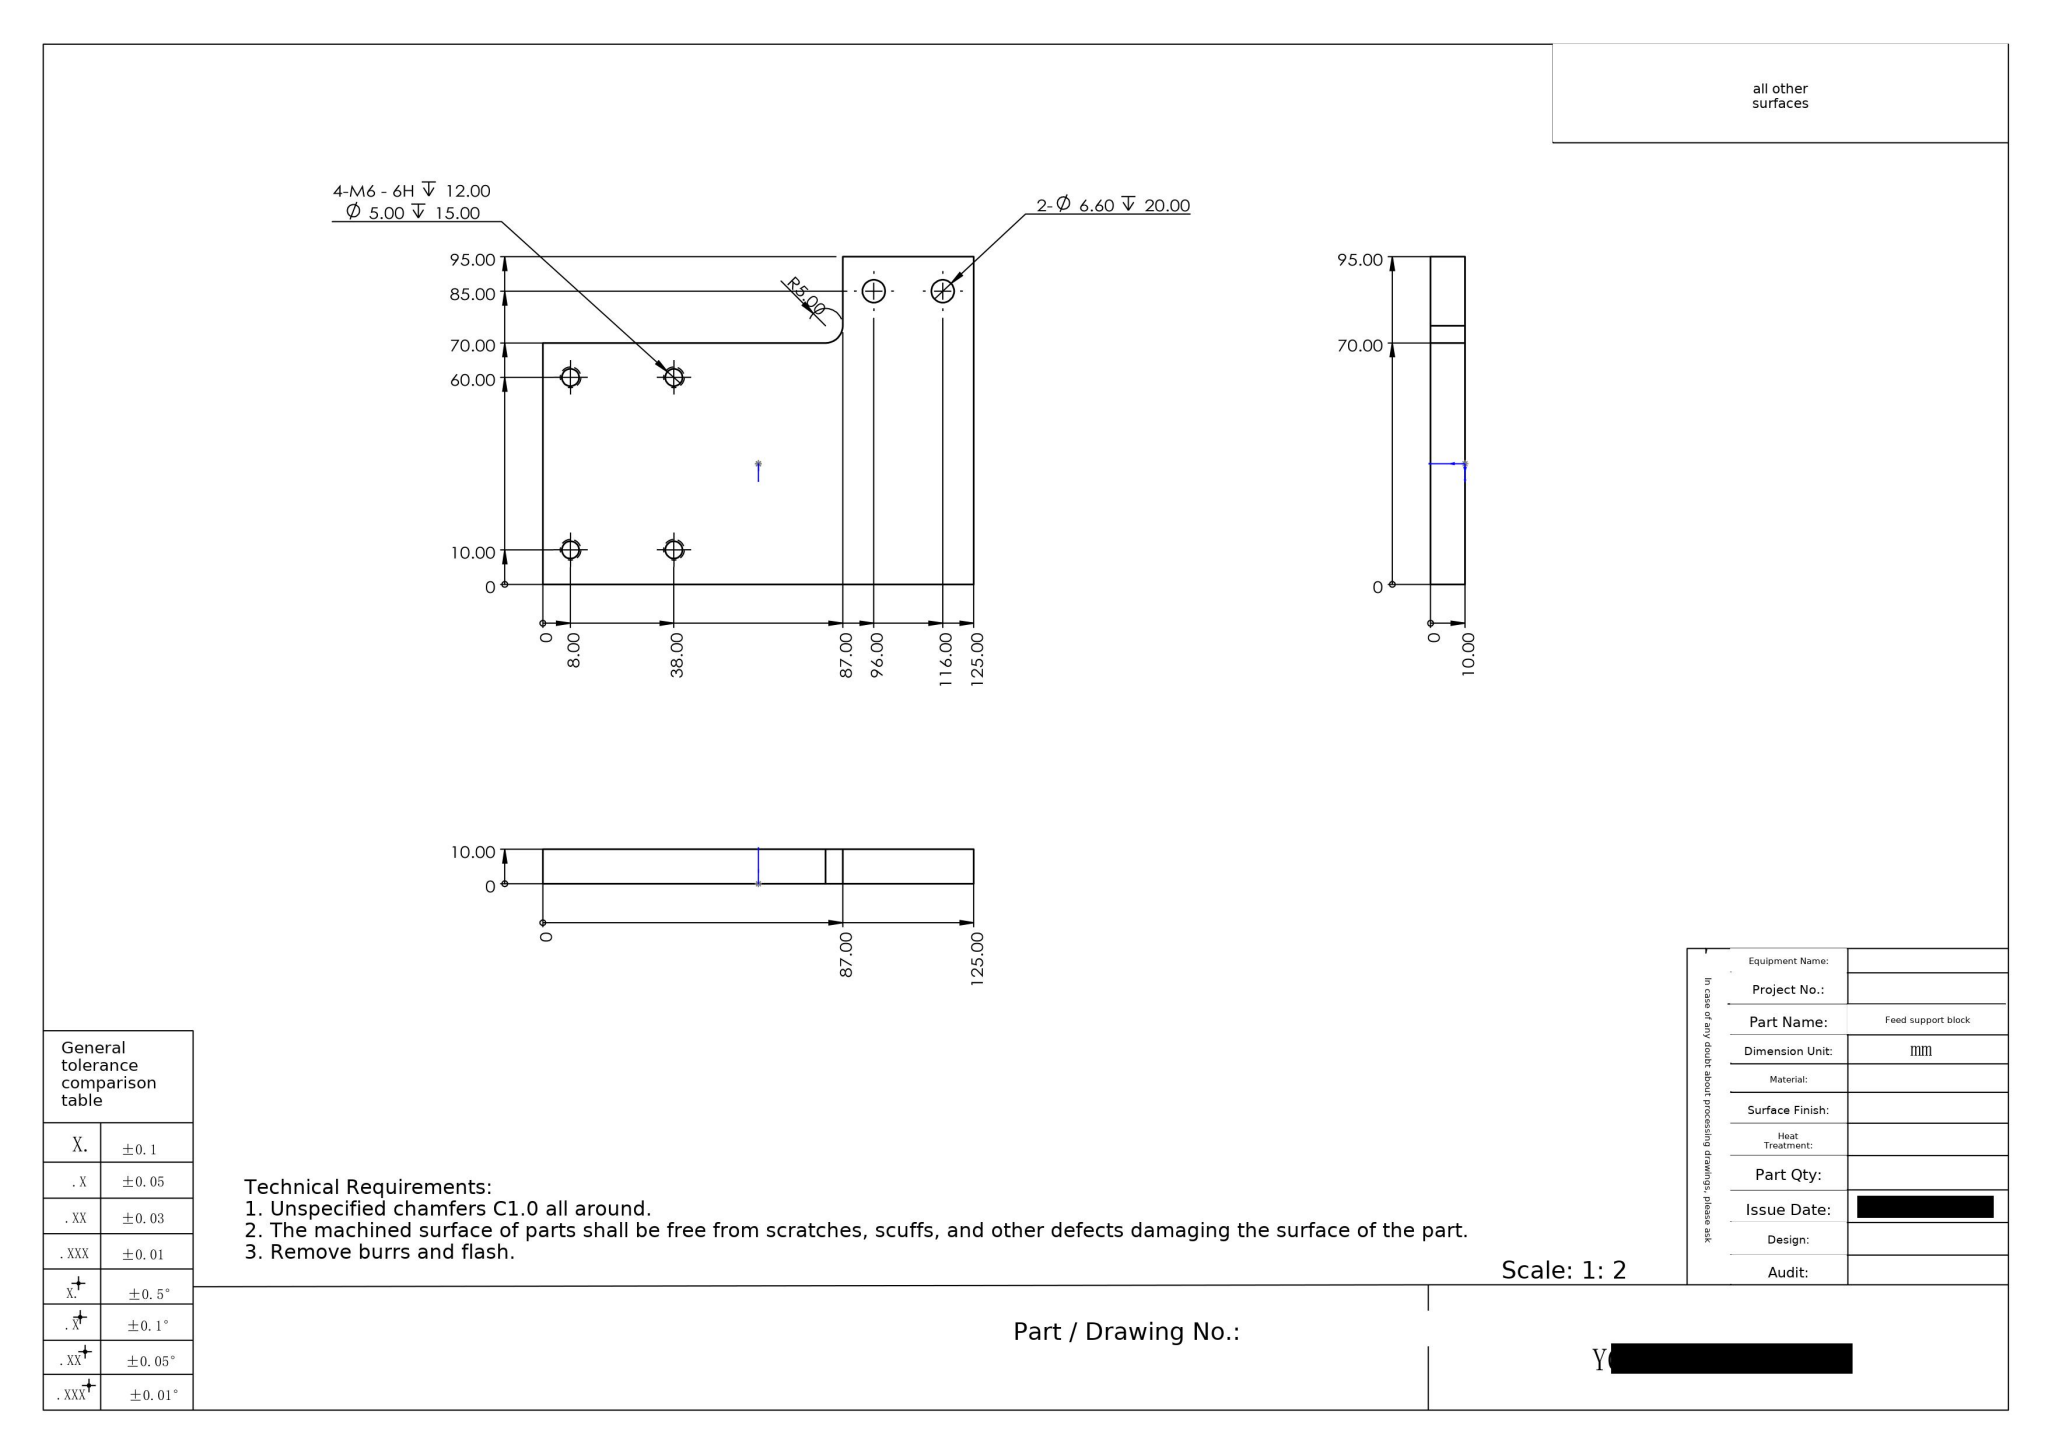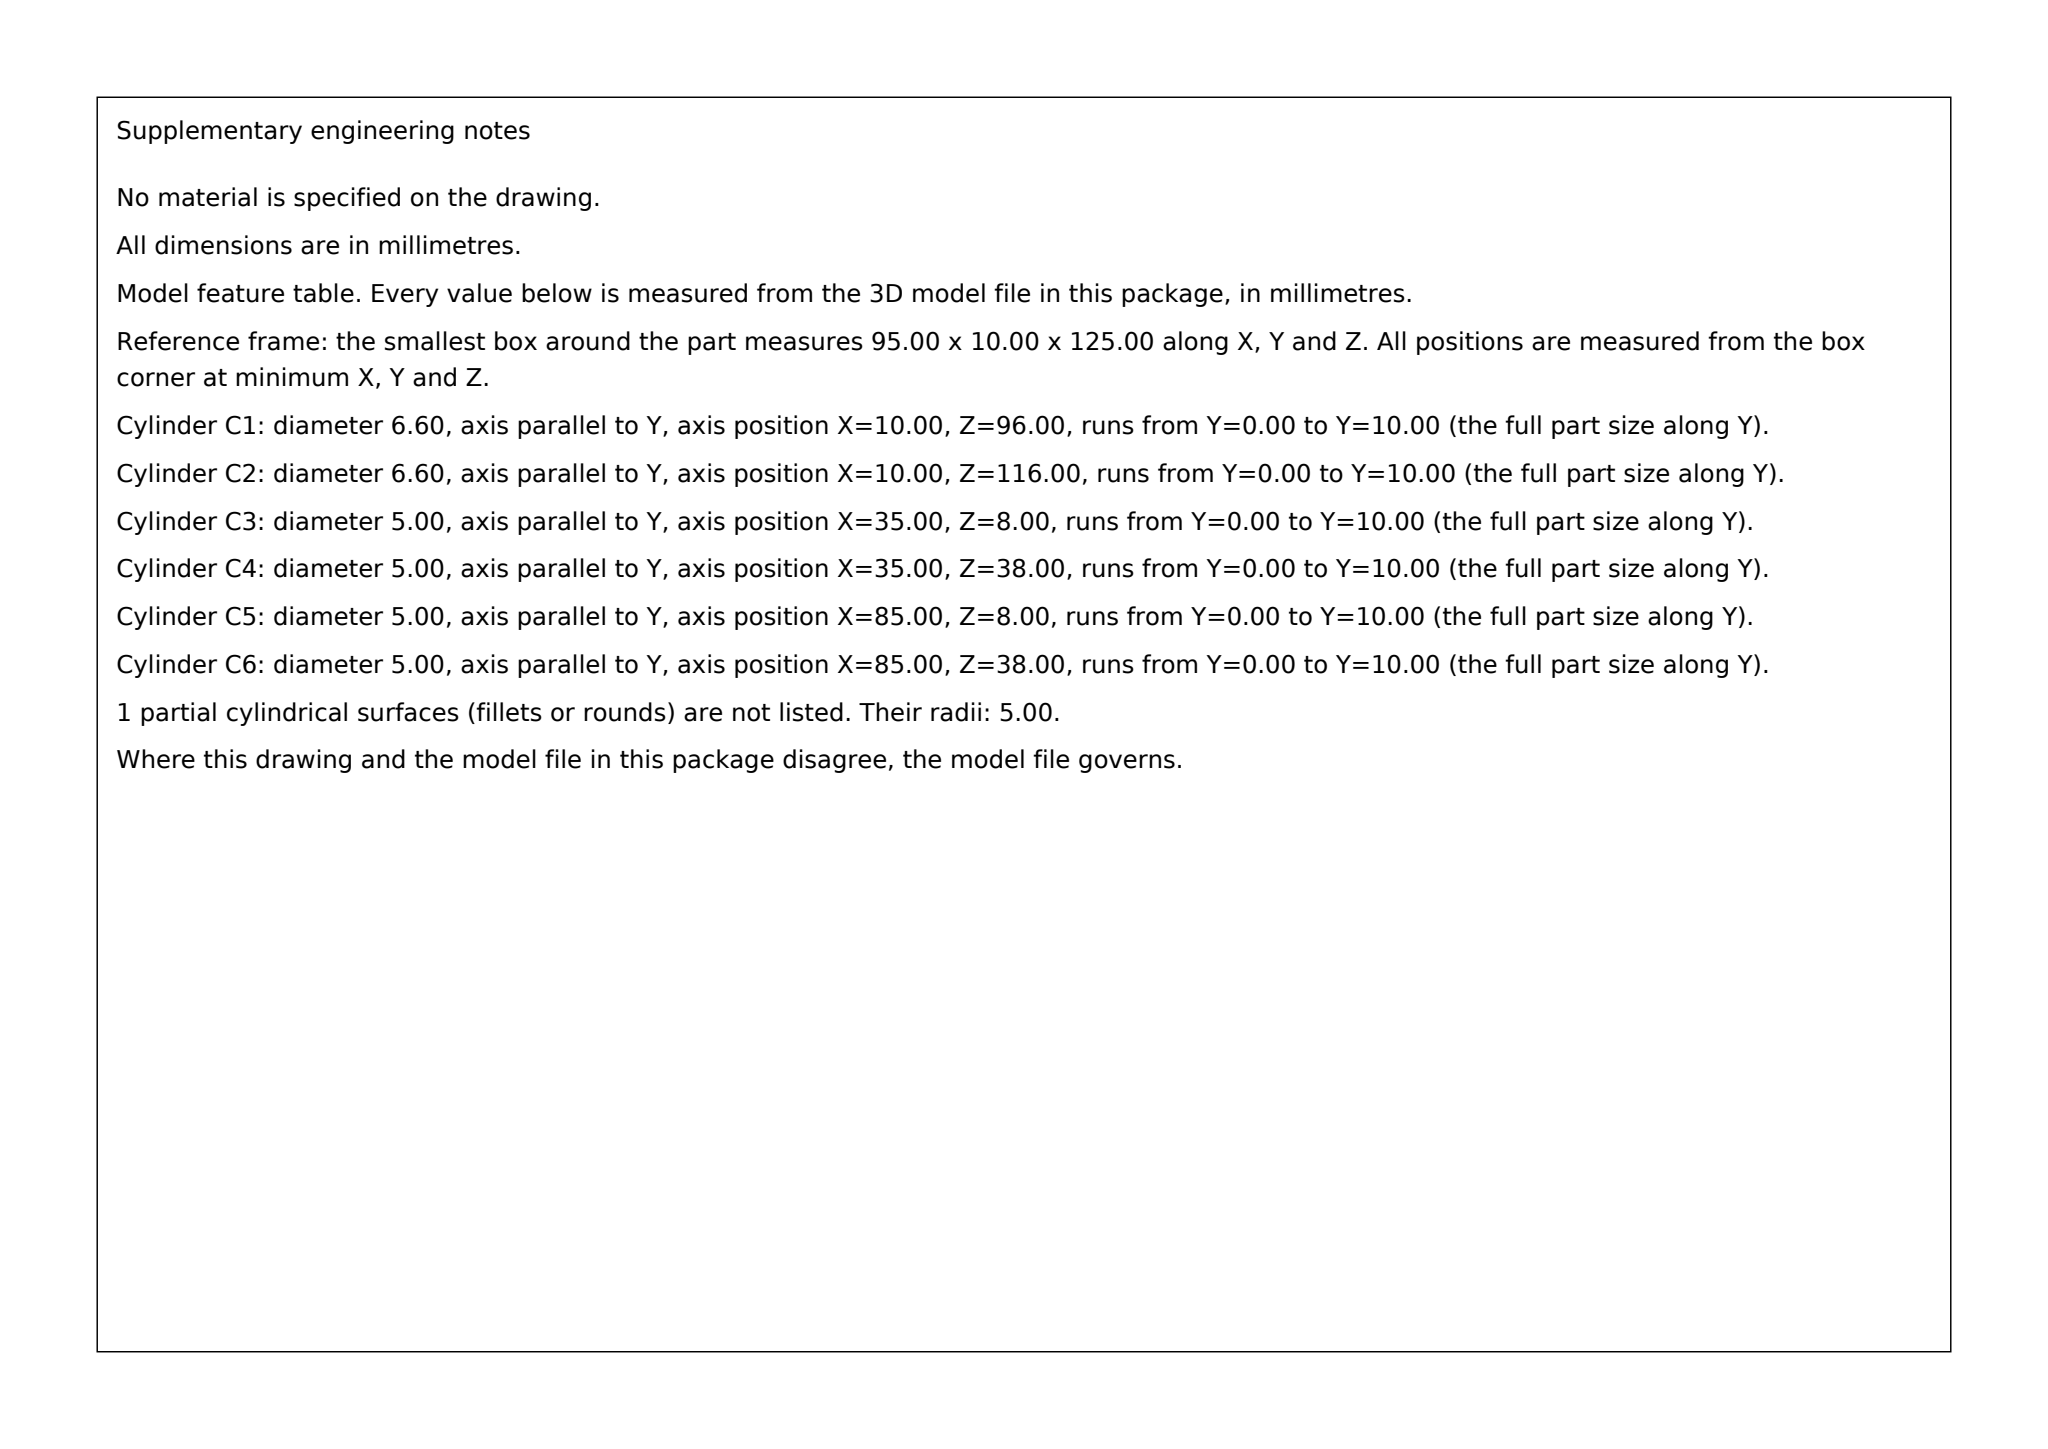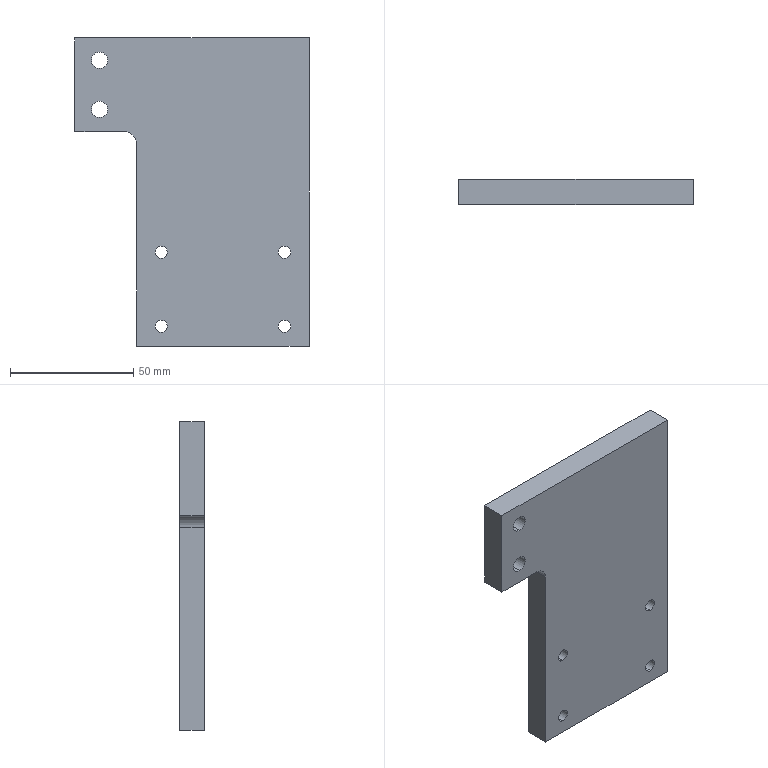Part | SolidWorks | mm | 1 solid | 21 faces | box 95 x 10 x 125 mm | volume 95584 mm3 | cylinder 13 | plane 8 | commonest cylinder face diameters 5 x8 6.6 x4 10 x1
build123d program:
from build123d import *

# Parameters (mm, degrees)
SKETCH1_W                = 70
SKETCH1_H                = 125
BOSS_EXTRUDE1_DEPTH      = 10
M6_TAPPED_HOLE1_D        = 5
M6_TAPPED_HOLE1_DEPTH    = 15
M6_TAPPED_HOLE1_TIP      = 1.502
SKETCH6_W                = 25
SKETCH6_H                = 38
BOSS_EXTRUDE2_DEPTH      = 10
M6_CLEARANCE_HOLE1_D     = 6.6
M6_CLEARANCE_HOLE1_DEPTH = 20
M6_CLEARANCE_HOLE1_TIP   = 1.983
FILLET1_R                = 5


with BuildPart() as part:
    # Sketch1 → Boss-Extrude1 (new body)
    with BuildSketch(Plane(origin=(0, 0, 0), x_dir=(1, 0, 0), z_dir=(0, 1, 0))):
        Rectangle(SKETCH1_W, SKETCH1_H)
    extrude(amount=BOSS_EXTRUDE1_DEPTH)

    # M6 Tapped Hole1
    with Locations(Plane(origin=(0, 10, 0), x_dir=(1, 0, 0), z_dir=(0, 1, 0))):
        with Locations((-25, 54.5), (25, 54.5), (-25, 24.5), (25, 24.5)):
            Hole(M6_TAPPED_HOLE1_D / 2, depth=M6_TAPPED_HOLE1_DEPTH)
            with Locations((0, 0, -(M6_TAPPED_HOLE1_DEPTH + M6_TAPPED_HOLE1_TIP / 2))):  # 118° drill point
                Cone(0, M6_TAPPED_HOLE1_D / 2, M6_TAPPED_HOLE1_TIP, mode=Mode.SUBTRACT)

    # Sketch6 → Boss-Extrude2 (add)
    with BuildSketch(Plane(origin=(0, 10, 0), x_dir=(1, 0, 0), z_dir=(0, 1, 0))):
        with Locations((-47.5, -43.5)):
            Rectangle(SKETCH6_W, SKETCH6_H)
    extrude(amount=-BOSS_EXTRUDE2_DEPTH)

    # M6 Clearance Hole1
    with Locations(Plane(origin=(0, 10, 0), x_dir=(1, 0, 0), z_dir=(0, 1, 0))):
        with Locations((-50, -33.5), (-50, -53.5)):
            Hole(M6_CLEARANCE_HOLE1_D / 2, depth=M6_CLEARANCE_HOLE1_DEPTH)
            with Locations((0, 0, -(M6_CLEARANCE_HOLE1_DEPTH + M6_CLEARANCE_HOLE1_TIP / 2))):  # 118° drill point
                Cone(0, M6_CLEARANCE_HOLE1_D / 2, M6_CLEARANCE_HOLE1_TIP, mode=Mode.SUBTRACT)

    # Fillet1
    fillet1_edges = [part.edges().sort_by_distance(p)[0] for p in [
        (-35, 5, 24.5),
    ]]
    fillet(fillet1_edges, radius=FILLET1_R)


solid = part.part
STEP:
#1=CARTESIAN_POINT('',(-50.,0.,30.2));
#2=VERTEX_POINT('',#1);
#3=CARTESIAN_POINT('',(-50.,0.,36.8));
#4=VERTEX_POINT('',#3);
#5=CARTESIAN_POINT('',(-50.,0.,33.5));
#6=DIRECTION('',(0.,1.,0.));
#7=DIRECTION('',(0.,0.,1.));
#8=AXIS2_PLACEMENT_3D('',#5,#6,#7);
#9=CIRCLE('',#8,3.3);
#10=EDGE_CURVE('',#2,#4,#9,.T.);
#11=ORIENTED_EDGE('',*,*,#10,.F.);
#12=CARTESIAN_POINT('',(-50.,10.,30.2));
#13=VERTEX_POINT('',#12);
#14=CARTESIAN_POINT('',(-50.,10.,30.2));
#15=DIRECTION('',(0.,1.,0.));
#16=VECTOR('',#15,1000.);
#17=LINE('',#14,#16);
#18=EDGE_CURVE('',#2,#13,#17,.T.);
#19=ORIENTED_EDGE('',*,*,#18,.T.);
#20=CARTESIAN_POINT('',(-50.,10.,36.8));
#21=VERTEX_POINT('',#20);
#22=CARTESIAN_POINT('',(-50.,10.,33.5));
#23=DIRECTION('',(0.,1.,0.));
#24=DIRECTION('',(0.,0.,1.));
#25=AXIS2_PLACEMENT_3D('',#22,#23,#24);
#26=CIRCLE('',#25,3.3);
#27=EDGE_CURVE('',#13,#21,#26,.T.);
#28=ORIENTED_EDGE('',*,*,#27,.T.);
#29=CARTESIAN_POINT('',(-50.,10.,36.8));
#30=DIRECTION('',(0.,1.,0.));
#31=VECTOR('',#30,1000.);
#32=LINE('',#29,#31);
#33=EDGE_CURVE('',#4,#21,#32,.T.);
#34=ORIENTED_EDGE('',*,*,#33,.F.);
#35=EDGE_LOOP('',(#11,#19,#28,#34));
#36=FACE_OUTER_BOUND('',#35,.T.);
#37=CARTESIAN_POINT('',(-50.,10.,33.5));
#38=DIRECTION('',(0.,1.,0.));
#39=DIRECTION('',(0.,0.,1.));
#40=AXIS2_PLACEMENT_3D('',#37,#38,#39);
#41=CYLINDRICAL_SURFACE('',#40,3.3);
#42=ADVANCED_FACE('',(#36),#41,.F.);
#43=CARTESIAN_POINT('',(-50.,0.,50.2));
#44=VERTEX_POINT('',#43);
#45=CARTESIAN_POINT('',(-50.,0.,56.8));
#46=VERTEX_POINT('',#45);
#47=CARTESIAN_POINT('',(-50.,0.,53.5));
#48=DIRECTION('',(0.,1.,0.));
#49=DIRECTION('',(0.,0.,1.));
#50=AXIS2_PLACEMENT_3D('',#47,#48,#49);
#51=CIRCLE('',#50,3.3);
#52=EDGE_CURVE('',#44,#46,#51,.T.);
#53=ORIENTED_EDGE('',*,*,#52,.F.);
#54=CARTESIAN_POINT('',(-50.,10.,50.2));
#55=VERTEX_POINT('',#54);
#56=CARTESIAN_POINT('',(-50.,10.,50.2));
#57=DIRECTION('',(0.,1.,0.));
#58=VECTOR('',#57,1000.);
#59=LINE('',#56,#58);
#60=EDGE_CURVE('',#44,#55,#59,.T.);
#61=ORIENTED_EDGE('',*,*,#60,.T.);
#62=CARTESIAN_POINT('',(-50.,10.,56.8));
#63=VERTEX_POINT('',#62);
#64=CARTESIAN_POINT('',(-50.,10.,53.5));
#65=DIRECTION('',(0.,1.,0.));
#66=DIRECTION('',(0.,0.,1.));
#67=AXIS2_PLACEMENT_3D('',#64,#65,#66);
#68=CIRCLE('',#67,3.3);
#69=EDGE_CURVE('',#55,#63,#68,.T.);
#70=ORIENTED_EDGE('',*,*,#69,.T.);
#71=CARTESIAN_POINT('',(-50.,10.,56.8));
#72=DIRECTION('',(0.,1.,0.));
#73=VECTOR('',#72,1000.);
#74=LINE('',#71,#73);
#75=EDGE_CURVE('',#46,#63,#74,.T.);
#76=ORIENTED_EDGE('',*,*,#75,.F.);
#77=EDGE_LOOP('',(#53,#61,#70,#76));
#78=FACE_OUTER_BOUND('',#77,.T.);
#79=CARTESIAN_POINT('',(-50.,10.,53.5));
#80=DIRECTION('',(0.,1.,0.));
#81=DIRECTION('',(0.,0.,1.));
#82=AXIS2_PLACEMENT_3D('',#79,#80,#81);
#83=CYLINDRICAL_SURFACE('',#82,3.3);
#84=ADVANCED_FACE('',(#78),#83,.F.);
#85=CARTESIAN_POINT('',(-25.,0.,-57.));
#86=VERTEX_POINT('',#85);
#87=CARTESIAN_POINT('',(-25.,0.,-52.));
#88=VERTEX_POINT('',#87);
#89=CARTESIAN_POINT('',(-25.,0.,-54.5));
#90=DIRECTION('',(0.,1.,0.));
#91=DIRECTION('',(0.,0.,1.));
#92=AXIS2_PLACEMENT_3D('',#89,#90,#91);
#93=CIRCLE('',#92,2.5);
#94=EDGE_CURVE('',#86,#88,#93,.T.);
#95=ORIENTED_EDGE('',*,*,#94,.F.);
#96=CARTESIAN_POINT('',(-25.,10.,-57.));
#97=VERTEX_POINT('',#96);
#98=CARTESIAN_POINT('',(-25.,10.,-57.));
#99=DIRECTION('',(0.,1.,0.));
#100=VECTOR('',#99,1000.);
#101=LINE('',#98,#100);
#102=EDGE_CURVE('',#86,#97,#101,.T.);
#103=ORIENTED_EDGE('',*,*,#102,.T.);
#104=CARTESIAN_POINT('',(-25.,10.,-52.));
#105=VERTEX_POINT('',#104);
#106=CARTESIAN_POINT('',(-25.,10.,-54.5));
#107=DIRECTION('',(0.,1.,0.));
#108=DIRECTION('',(0.,0.,1.));
#109=AXIS2_PLACEMENT_3D('',#106,#107,#108);
#110=CIRCLE('',#109,2.5);
#111=EDGE_CURVE('',#97,#105,#110,.T.);
#112=ORIENTED_EDGE('',*,*,#111,.T.);
#113=CARTESIAN_POINT('',(-25.,10.,-52.));
#114=DIRECTION('',(0.,1.,0.));
#115=VECTOR('',#114,1000.);
#116=LINE('',#113,#115);
#117=EDGE_CURVE('',#88,#105,#116,.T.);
#118=ORIENTED_EDGE('',*,*,#117,.F.);
#119=EDGE_LOOP('',(#95,#103,#112,#118));
#120=FACE_OUTER_BOUND('',#119,.T.);
#121=CARTESIAN_POINT('',(-25.,10.,-54.5));
#122=DIRECTION('',(0.,1.,0.));
#123=DIRECTION('',(0.,0.,1.));
#124=AXIS2_PLACEMENT_3D('',#121,#122,#123);
#125=CYLINDRICAL_SURFACE('',#124,2.5);
#126=ADVANCED_FACE('',(#120),#125,.F.);
#127=CARTESIAN_POINT('',(25.,0.,-57.));
#128=VERTEX_POINT('',#127);
#129=CARTESIAN_POINT('',(25.,0.,-52.));
#130=VERTEX_POINT('',#129);
#131=CARTESIAN_POINT('',(25.,0.,-54.5));
#132=DIRECTION('',(0.,1.,0.));
#133=DIRECTION('',(0.,0.,1.));
#134=AXIS2_PLACEMENT_3D('',#131,#132,#133);
#135=CIRCLE('',#134,2.5);
#136=EDGE_CURVE('',#128,#130,#135,.T.);
#137=ORIENTED_EDGE('',*,*,#136,.F.);
#138=CARTESIAN_POINT('',(25.,10.,-57.));
#139=VERTEX_POINT('',#138);
#140=CARTESIAN_POINT('',(25.,10.,-57.));
#141=DIRECTION('',(0.,1.,0.));
#142=VECTOR('',#141,1000.);
#143=LINE('',#140,#142);
#144=EDGE_CURVE('',#128,#139,#143,.T.);
#145=ORIENTED_EDGE('',*,*,#144,.T.);
#146=CARTESIAN_POINT('',(25.,10.,-52.));
#147=VERTEX_POINT('',#146);
#148=CARTESIAN_POINT('',(25.,10.,-54.5));
#149=DIRECTION('',(0.,1.,0.));
#150=DIRECTION('',(0.,0.,1.));
#151=AXIS2_PLACEMENT_3D('',#148,#149,#150);
#152=CIRCLE('',#151,2.5);
#153=EDGE_CURVE('',#139,#147,#152,.T.);
#154=ORIENTED_EDGE('',*,*,#153,.T.);
#155=CARTESIAN_POINT('',(25.,10.,-52.));
#156=DIRECTION('',(0.,1.,0.));
#157=VECTOR('',#156,1000.);
#158=LINE('',#155,#157);
#159=EDGE_CURVE('',#130,#147,#158,.T.);
#160=ORIENTED_EDGE('',*,*,#159,.F.);
#161=EDGE_LOOP('',(#137,#145,#154,#160));
#162=FACE_OUTER_BOUND('',#161,.T.);
#163=CARTESIAN_POINT('',(25.,10.,-54.5));
#164=DIRECTION('',(0.,1.,0.));
#165=DIRECTION('',(0.,0.,1.));
#166=AXIS2_PLACEMENT_3D('',#163,#164,#165);
#167=CYLINDRICAL_SURFACE('',#166,2.5);
#168=ADVANCED_FACE('',(#162),#167,.F.);
#169=CARTESIAN_POINT('',(-25.,0.,-27.));
#170=VERTEX_POINT('',#169);
#171=CARTESIAN_POINT('',(-25.,0.,-22.));
#172=VERTEX_POINT('',#171);
#173=CARTESIAN_POINT('',(-25.,0.,-24.5));
#174=DIRECTION('',(0.,1.,0.));
#175=DIRECTION('',(0.,0.,1.));
#176=AXIS2_PLACEMENT_3D('',#173,#174,#175);
#177=CIRCLE('',#176,2.5);
#178=EDGE_CURVE('',#170,#172,#177,.T.);
#179=ORIENTED_EDGE('',*,*,#178,.F.);
#180=CARTESIAN_POINT('',(-25.,10.,-27.));
#181=VERTEX_POINT('',#180);
#182=CARTESIAN_POINT('',(-25.,10.,-27.));
#183=DIRECTION('',(0.,1.,0.));
#184=VECTOR('',#183,1000.);
#185=LINE('',#182,#184);
#186=EDGE_CURVE('',#170,#181,#185,.T.);
#187=ORIENTED_EDGE('',*,*,#186,.T.);
#188=CARTESIAN_POINT('',(-25.,10.,-22.));
#189=VERTEX_POINT('',#188);
#190=CARTESIAN_POINT('',(-25.,10.,-24.5));
#191=DIRECTION('',(0.,1.,0.));
#192=DIRECTION('',(0.,0.,1.));
#193=AXIS2_PLACEMENT_3D('',#190,#191,#192);
#194=CIRCLE('',#193,2.5);
#195=EDGE_CURVE('',#181,#189,#194,.T.);
#196=ORIENTED_EDGE('',*,*,#195,.T.);
#197=CARTESIAN_POINT('',(-25.,10.,-22.));
#198=DIRECTION('',(0.,1.,0.));
#199=VECTOR('',#198,1000.);
#200=LINE('',#197,#199);
#201=EDGE_CURVE('',#172,#189,#200,.T.);
#202=ORIENTED_EDGE('',*,*,#201,.F.);
#203=EDGE_LOOP('',(#179,#187,#196,#202));
#204=FACE_OUTER_BOUND('',#203,.T.);
#205=CARTESIAN_POINT('',(-25.,10.,-24.5));
#206=DIRECTION('',(0.,1.,0.));
#207=DIRECTION('',(0.,0.,1.));
#208=AXIS2_PLACEMENT_3D('',#205,#206,#207);
#209=CYLINDRICAL_SURFACE('',#208,2.5);
#210=ADVANCED_FACE('',(#204),#209,.F.);
#211=CARTESIAN_POINT('',(25.,0.,-27.));
#212=VERTEX_POINT('',#211);
#213=CARTESIAN_POINT('',(25.,0.,-22.));
#214=VERTEX_POINT('',#213);
#215=CARTESIAN_POINT('',(25.,0.,-24.5));
#216=DIRECTION('',(0.,1.,0.));
#217=DIRECTION('',(0.,0.,1.));
#218=AXIS2_PLACEMENT_3D('',#215,#216,#217);
#219=CIRCLE('',#218,2.5);
#220=EDGE_CURVE('',#212,#214,#219,.T.);
#221=ORIENTED_EDGE('',*,*,#220,.F.);
#222=CARTESIAN_POINT('',(25.,10.,-27.));
#223=VERTEX_POINT('',#222);
#224=CARTESIAN_POINT('',(25.,10.,-27.));
#225=DIRECTION('',(0.,1.,0.));
#226=VECTOR('',#225,1000.);
#227=LINE('',#224,#226);
#228=EDGE_CURVE('',#212,#223,#227,.T.);
#229=ORIENTED_EDGE('',*,*,#228,.T.);
#230=CARTESIAN_POINT('',(25.,10.,-22.));
#231=VERTEX_POINT('',#230);
#232=CARTESIAN_POINT('',(25.,10.,-24.5));
#233=DIRECTION('',(0.,1.,0.));
#234=DIRECTION('',(0.,0.,1.));
#235=AXIS2_PLACEMENT_3D('',#232,#233,#234);
#236=CIRCLE('',#235,2.5);
#237=EDGE_CURVE('',#223,#231,#236,.T.);
#238=ORIENTED_EDGE('',*,*,#237,.T.);
#239=CARTESIAN_POINT('',(25.,10.,-22.));
#240=DIRECTION('',(0.,1.,0.));
#241=VECTOR('',#240,1000.);
#242=LINE('',#239,#241);
#243=EDGE_CURVE('',#214,#231,#242,.T.);
#244=ORIENTED_EDGE('',*,*,#243,.F.);
#245=EDGE_LOOP('',(#221,#229,#238,#244));
#246=FACE_OUTER_BOUND('',#245,.T.);
#247=CARTESIAN_POINT('',(25.,10.,-24.5));
#248=DIRECTION('',(0.,1.,0.));
#249=DIRECTION('',(0.,0.,1.));
#250=AXIS2_PLACEMENT_3D('',#247,#248,#249);
#251=CYLINDRICAL_SURFACE('',#250,2.5);
#252=ADVANCED_FACE('',(#246),#251,.F.);
#253=CARTESIAN_POINT('',(-35.,0.,-62.5));
#254=VERTEX_POINT('',#253);
#255=CARTESIAN_POINT('',(-35.,0.,19.5));
#256=VERTEX_POINT('',#255);
#257=CARTESIAN_POINT('',(-35.,0.,-62.5));
#258=DIRECTION('',(0.,0.,1.));
#259=VECTOR('',#258,1000.);
#260=LINE('',#257,#259);
#261=EDGE_CURVE('',#254,#256,#260,.T.);
#262=ORIENTED_EDGE('',*,*,#261,.T.);
#263=CARTESIAN_POINT('',(-35.,10.,19.5));
#264=VERTEX_POINT('',#263);
#265=CARTESIAN_POINT('',(-35.,10.,19.5));
#266=DIRECTION('',(0.,1.,0.));
#267=VECTOR('',#266,1000.);
#268=LINE('',#265,#267);
#269=EDGE_CURVE('',#256,#264,#268,.T.);
#270=ORIENTED_EDGE('',*,*,#269,.T.);
#271=CARTESIAN_POINT('',(-35.,10.,-62.5));
#272=VERTEX_POINT('',#271);
#273=CARTESIAN_POINT('',(-35.,10.,-62.5));
#274=DIRECTION('',(0.,0.,1.));
#275=VECTOR('',#274,1000.);
#276=LINE('',#273,#275);
#277=EDGE_CURVE('',#272,#264,#276,.T.);
#278=ORIENTED_EDGE('',*,*,#277,.F.);
#279=CARTESIAN_POINT('',(-35.,10.,-62.5));
#280=DIRECTION('',(0.,-1.,0.));
#281=VECTOR('',#280,1000.);
#282=LINE('',#279,#281);
#283=EDGE_CURVE('',#272,#254,#282,.T.);
#284=ORIENTED_EDGE('',*,*,#283,.T.);
#285=EDGE_LOOP('',(#262,#270,#278,#284));
#286=FACE_OUTER_BOUND('',#285,.T.);
#287=CARTESIAN_POINT('',(-35.,10.,-62.5));
#288=DIRECTION('',(1.,0.,-0.));
#289=DIRECTION('',(-0.,0.,-1.));
#290=AXIS2_PLACEMENT_3D('',#287,#288,#289);
#291=PLANE('',#290);
#292=ADVANCED_FACE('',(#286),#291,.F.);
#293=CARTESIAN_POINT('',(-60.,0.,62.5));
#294=VERTEX_POINT('',#293);
#295=CARTESIAN_POINT('',(35.,0.,62.5));
#296=VERTEX_POINT('',#295);
#297=CARTESIAN_POINT('',(-35.,0.,62.5));
#298=DIRECTION('',(1.,0.,0.));
#299=VECTOR('',#298,1000.);
#300=LINE('',#297,#299);
#301=EDGE_CURVE('',#294,#296,#300,.T.);
#302=ORIENTED_EDGE('',*,*,#301,.T.);
#303=CARTESIAN_POINT('',(35.,10.,62.5));
#304=VERTEX_POINT('',#303);
#305=CARTESIAN_POINT('',(35.,10.,62.5));
#306=DIRECTION('',(0.,-1.,0.));
#307=VECTOR('',#306,1000.);
#308=LINE('',#305,#307);
#309=EDGE_CURVE('',#304,#296,#308,.T.);
#310=ORIENTED_EDGE('',*,*,#309,.F.);
#311=CARTESIAN_POINT('',(-60.,10.,62.5));
#312=VERTEX_POINT('',#311);
#313=CARTESIAN_POINT('',(-35.,10.,62.5));
#314=DIRECTION('',(1.,0.,0.));
#315=VECTOR('',#314,1000.);
#316=LINE('',#313,#315);
#317=EDGE_CURVE('',#312,#304,#316,.T.);
#318=ORIENTED_EDGE('',*,*,#317,.F.);
#319=CARTESIAN_POINT('',(-60.,-45.486,62.5));
#320=DIRECTION('',(0.,1.,0.));
#321=VECTOR('',#320,1000.);
#322=LINE('',#319,#321);
#323=EDGE_CURVE('',#294,#312,#322,.T.);
#324=ORIENTED_EDGE('',*,*,#323,.F.);
#325=EDGE_LOOP('',(#302,#310,#318,#324));
#326=FACE_OUTER_BOUND('',#325,.T.);
#327=CARTESIAN_POINT('',(-35.,10.,62.5));
#328=DIRECTION('',(0.,0.,-1.));
#329=DIRECTION('',(-1.,0.,0.));
#330=AXIS2_PLACEMENT_3D('',#327,#328,#329);
#331=PLANE('',#330);
#332=ADVANCED_FACE('',(#326),#331,.F.);
#333=CARTESIAN_POINT('',(35.,0.,-62.5));
#334=VERTEX_POINT('',#333);
#335=CARTESIAN_POINT('',(35.,0.,-62.5));
#336=DIRECTION('',(0.,0.,1.));
#337=VECTOR('',#336,1000.);
#338=LINE('',#335,#337);
#339=EDGE_CURVE('',#334,#296,#338,.T.);
#340=ORIENTED_EDGE('',*,*,#339,.F.);
#341=CARTESIAN_POINT('',(35.,10.,-62.5));
#342=VERTEX_POINT('',#341);
#343=CARTESIAN_POINT('',(35.,10.,-62.5));
#344=DIRECTION('',(0.,-1.,0.));
#345=VECTOR('',#344,1000.);
#346=LINE('',#343,#345);
#347=EDGE_CURVE('',#342,#334,#346,.T.);
#348=ORIENTED_EDGE('',*,*,#347,.F.);
#349=CARTESIAN_POINT('',(35.,10.,-62.5));
#350=DIRECTION('',(0.,0.,1.));
#351=VECTOR('',#350,1000.);
#352=LINE('',#349,#351);
#353=EDGE_CURVE('',#342,#304,#352,.T.);
#354=ORIENTED_EDGE('',*,*,#353,.T.);
#355=ORIENTED_EDGE('',*,*,#309,.T.);
#356=EDGE_LOOP('',(#340,#348,#354,#355));
#357=FACE_OUTER_BOUND('',#356,.T.);
#358=CARTESIAN_POINT('',(35.,10.,-62.5));
#359=DIRECTION('',(1.,0.,-0.));
#360=DIRECTION('',(-0.,0.,-1.));
#361=AXIS2_PLACEMENT_3D('',#358,#359,#360);
#362=PLANE('',#361);
#363=ADVANCED_FACE('',(#357),#362,.T.);
#364=CARTESIAN_POINT('',(-35.,0.,-62.5));
#365=DIRECTION('',(1.,0.,0.));
#366=VECTOR('',#365,1000.);
#367=LINE('',#364,#366);
#368=EDGE_CURVE('',#254,#334,#367,.T.);
#369=ORIENTED_EDGE('',*,*,#368,.F.);
#370=ORIENTED_EDGE('',*,*,#283,.F.);
#371=CARTESIAN_POINT('',(-35.,10.,-62.5));
#372=DIRECTION('',(1.,0.,0.));
#373=VECTOR('',#372,1000.);
#374=LINE('',#371,#373);
#375=EDGE_CURVE('',#272,#342,#374,.T.);
#376=ORIENTED_EDGE('',*,*,#375,.T.);
#377=ORIENTED_EDGE('',*,*,#347,.T.);
#378=EDGE_LOOP('',(#369,#370,#376,#377));
#379=FACE_OUTER_BOUND('',#378,.T.);
#380=CARTESIAN_POINT('',(-35.,10.,-62.5));
#381=DIRECTION('',(0.,0.,-1.));
#382=DIRECTION('',(-1.,0.,0.));
#383=AXIS2_PLACEMENT_3D('',#380,#381,#382);
#384=PLANE('',#383);
#385=ADVANCED_FACE('',(#379),#384,.T.);
#386=CARTESIAN_POINT('',(-50.,10.,33.5));
#387=DIRECTION('',(0.,1.,0.));
#388=DIRECTION('',(0.,0.,1.));
#389=AXIS2_PLACEMENT_3D('',#386,#387,#388);
#390=CIRCLE('',#389,3.3);
#391=EDGE_CURVE('',#21,#13,#390,.T.);
#392=ORIENTED_EDGE('',*,*,#391,.F.);
#393=ORIENTED_EDGE('',*,*,#27,.F.);
#394=EDGE_LOOP('',(#392,#393));
#395=FACE_BOUND('',#394,.T.);
#396=CARTESIAN_POINT('',(-50.,10.,53.5));
#397=DIRECTION('',(0.,1.,0.));
#398=DIRECTION('',(0.,0.,1.));
#399=AXIS2_PLACEMENT_3D('',#396,#397,#398);
#400=CIRCLE('',#399,3.3);
#401=EDGE_CURVE('',#63,#55,#400,.T.);
#402=ORIENTED_EDGE('',*,*,#401,.F.);
#403=ORIENTED_EDGE('',*,*,#69,.F.);
#404=EDGE_LOOP('',(#402,#403));
#405=FACE_BOUND('',#404,.T.);
#406=CARTESIAN_POINT('',(-25.,10.,-54.5));
#407=DIRECTION('',(0.,1.,0.));
#408=DIRECTION('',(0.,0.,1.));
#409=AXIS2_PLACEMENT_3D('',#406,#407,#408);
#410=CIRCLE('',#409,2.5);
#411=EDGE_CURVE('',#105,#97,#410,.T.);
#412=ORIENTED_EDGE('',*,*,#411,.F.);
#413=ORIENTED_EDGE('',*,*,#111,.F.);
#414=EDGE_LOOP('',(#412,#413));
#415=FACE_BOUND('',#414,.T.);
#416=CARTESIAN_POINT('',(25.,10.,-54.5));
#417=DIRECTION('',(0.,1.,0.));
#418=DIRECTION('',(0.,0.,1.));
#419=AXIS2_PLACEMENT_3D('',#416,#417,#418);
#420=CIRCLE('',#419,2.5);
#421=EDGE_CURVE('',#147,#139,#420,.T.);
#422=ORIENTED_EDGE('',*,*,#421,.F.);
#423=ORIENTED_EDGE('',*,*,#153,.F.);
#424=EDGE_LOOP('',(#422,#423));
#425=FACE_BOUND('',#424,.T.);
#426=CARTESIAN_POINT('',(-25.,10.,-24.5));
#427=DIRECTION('',(0.,1.,0.));
#428=DIRECTION('',(0.,0.,1.));
#429=AXIS2_PLACEMENT_3D('',#426,#427,#428);
#430=CIRCLE('',#429,2.5);
#431=EDGE_CURVE('',#189,#181,#430,.T.);
#432=ORIENTED_EDGE('',*,*,#431,.F.);
#433=ORIENTED_EDGE('',*,*,#195,.F.);
#434=EDGE_LOOP('',(#432,#433));
#435=FACE_BOUND('',#434,.T.);
#436=CARTESIAN_POINT('',(25.,10.,-24.5));
#437=DIRECTION('',(0.,1.,0.));
#438=DIRECTION('',(0.,0.,1.));
#439=AXIS2_PLACEMENT_3D('',#436,#437,#438);
#440=CIRCLE('',#439,2.5);
#441=EDGE_CURVE('',#231,#223,#440,.T.);
#442=ORIENTED_EDGE('',*,*,#441,.F.);
#443=ORIENTED_EDGE('',*,*,#237,.F.);
#444=EDGE_LOOP('',(#442,#443));
#445=FACE_BOUND('',#444,.T.);
#446=ORIENTED_EDGE('',*,*,#277,.T.);
#447=CARTESIAN_POINT('',(-40.,10.,24.5));
#448=VERTEX_POINT('',#447);
#449=CARTESIAN_POINT('',(-40.,10.,19.5));
#450=DIRECTION('',(0.,-1.,0.));
#451=DIRECTION('',(0.,0.,1.));
#452=AXIS2_PLACEMENT_3D('',#449,#450,#451);
#453=CIRCLE('',#452,5.);
#454=EDGE_CURVE('',#264,#448,#453,.T.);
#455=ORIENTED_EDGE('',*,*,#454,.T.);
#456=CARTESIAN_POINT('',(-60.,10.,24.5));
#457=VERTEX_POINT('',#456);
#458=CARTESIAN_POINT('',(-35.,10.,24.5));
#459=DIRECTION('',(-1.,0.,0.));
#460=VECTOR('',#459,1000.);
#461=LINE('',#458,#460);
#462=EDGE_CURVE('',#448,#457,#461,.T.);
#463=ORIENTED_EDGE('',*,*,#462,.T.);
#464=CARTESIAN_POINT('',(-60.,10.,24.5));
#465=DIRECTION('',(0.,0.,1.));
#466=VECTOR('',#465,1000.);
#467=LINE('',#464,#466);
#468=EDGE_CURVE('',#457,#312,#467,.T.);
#469=ORIENTED_EDGE('',*,*,#468,.T.);
#470=ORIENTED_EDGE('',*,*,#317,.T.);
#471=ORIENTED_EDGE('',*,*,#353,.F.);
#472=ORIENTED_EDGE('',*,*,#375,.F.);
#473=EDGE_LOOP('',(#446,#455,#463,#469,#470,#471,#472));
#474=FACE_OUTER_BOUND('',#473,.T.);
#475=CARTESIAN_POINT('',(0.,10.,0.));
#476=DIRECTION('',(0.,1.,0.));
#477=DIRECTION('',(0.,0.,1.));
#478=AXIS2_PLACEMENT_3D('',#475,#476,#477);
#479=PLANE('',#478);
#480=ADVANCED_FACE('',(#395,#405,#415,#425,#435,#445,#474),#479,.T.);
#481=CARTESIAN_POINT('',(-50.,0.,33.5));
#482=DIRECTION('',(0.,1.,0.));
#483=DIRECTION('',(0.,0.,1.));
#484=AXIS2_PLACEMENT_3D('',#481,#482,#483);
#485=CIRCLE('',#484,3.3);
#486=EDGE_CURVE('',#4,#2,#485,.T.);
#487=ORIENTED_EDGE('',*,*,#486,.T.);
#488=ORIENTED_EDGE('',*,*,#10,.T.);
#489=EDGE_LOOP('',(#487,#488));
#490=FACE_BOUND('',#489,.T.);
#491=CARTESIAN_POINT('',(-50.,0.,53.5));
#492=DIRECTION('',(0.,1.,0.));
#493=DIRECTION('',(0.,0.,1.));
#494=AXIS2_PLACEMENT_3D('',#491,#492,#493);
#495=CIRCLE('',#494,3.3);
#496=EDGE_CURVE('',#46,#44,#495,.T.);
#497=ORIENTED_EDGE('',*,*,#496,.T.);
#498=ORIENTED_EDGE('',*,*,#52,.T.);
#499=EDGE_LOOP('',(#497,#498));
#500=FACE_BOUND('',#499,.T.);
#501=CARTESIAN_POINT('',(-25.,0.,-54.5));
#502=DIRECTION('',(0.,1.,0.));
#503=DIRECTION('',(0.,0.,1.));
#504=AXIS2_PLACEMENT_3D('',#501,#502,#503);
#505=CIRCLE('',#504,2.5);
#506=EDGE_CURVE('',#88,#86,#505,.T.);
#507=ORIENTED_EDGE('',*,*,#506,.T.);
#508=ORIENTED_EDGE('',*,*,#94,.T.);
#509=EDGE_LOOP('',(#507,#508));
#510=FACE_BOUND('',#509,.T.);
#511=CARTESIAN_POINT('',(25.,0.,-54.5));
#512=DIRECTION('',(0.,1.,0.));
#513=DIRECTION('',(0.,0.,1.));
#514=AXIS2_PLACEMENT_3D('',#511,#512,#513);
#515=CIRCLE('',#514,2.5);
#516=EDGE_CURVE('',#130,#128,#515,.T.);
#517=ORIENTED_EDGE('',*,*,#516,.T.);
#518=ORIENTED_EDGE('',*,*,#136,.T.);
#519=EDGE_LOOP('',(#517,#518));
#520=FACE_BOUND('',#519,.T.);
#521=CARTESIAN_POINT('',(-25.,0.,-24.5));
#522=DIRECTION('',(0.,1.,0.));
#523=DIRECTION('',(0.,0.,1.));
#524=AXIS2_PLACEMENT_3D('',#521,#522,#523);
#525=CIRCLE('',#524,2.5);
#526=EDGE_CURVE('',#172,#170,#525,.T.);
#527=ORIENTED_EDGE('',*,*,#526,.T.);
#528=ORIENTED_EDGE('',*,*,#178,.T.);
#529=EDGE_LOOP('',(#527,#528));
#530=FACE_BOUND('',#529,.T.);
#531=CARTESIAN_POINT('',(25.,0.,-24.5));
#532=DIRECTION('',(0.,1.,0.));
#533=DIRECTION('',(0.,0.,1.));
#534=AXIS2_PLACEMENT_3D('',#531,#532,#533);
#535=CIRCLE('',#534,2.5);
#536=EDGE_CURVE('',#214,#212,#535,.T.);
#537=ORIENTED_EDGE('',*,*,#536,.T.);
#538=ORIENTED_EDGE('',*,*,#220,.T.);
#539=EDGE_LOOP('',(#537,#538));
#540=FACE_BOUND('',#539,.T.);
#541=ORIENTED_EDGE('',*,*,#261,.F.);
#542=ORIENTED_EDGE('',*,*,#368,.T.);
#543=ORIENTED_EDGE('',*,*,#339,.T.);
#544=ORIENTED_EDGE('',*,*,#301,.F.);
#545=CARTESIAN_POINT('',(-60.,0.,24.5));
#546=VERTEX_POINT('',#545);
#547=CARTESIAN_POINT('',(-60.,0.,24.5));
#548=DIRECTION('',(-0.,0.,-1.));
#549=VECTOR('',#548,1000.);
#550=LINE('',#547,#549);
#551=EDGE_CURVE('',#294,#546,#550,.T.);
#552=ORIENTED_EDGE('',*,*,#551,.T.);
#553=CARTESIAN_POINT('',(-40.,0.,24.5));
#554=VERTEX_POINT('',#553);
#555=CARTESIAN_POINT('',(-35.,0.,24.5));
#556=DIRECTION('',(1.,0.,-0.));
#557=VECTOR('',#556,1000.);
#558=LINE('',#555,#557);
#559=EDGE_CURVE('',#546,#554,#558,.T.);
#560=ORIENTED_EDGE('',*,*,#559,.T.);
#561=CARTESIAN_POINT('',(-40.,0.,19.5));
#562=DIRECTION('',(0.,1.,0.));
#563=DIRECTION('',(0.,0.,1.));
#564=AXIS2_PLACEMENT_3D('',#561,#562,#563);
#565=CIRCLE('',#564,5.);
#566=EDGE_CURVE('',#554,#256,#565,.T.);
#567=ORIENTED_EDGE('',*,*,#566,.T.);
#568=EDGE_LOOP('',(#541,#542,#543,#544,#552,#560,#567));
#569=FACE_OUTER_BOUND('',#568,.T.);
#570=CARTESIAN_POINT('',(0.,0.,0.));
#571=DIRECTION('',(0.,1.,0.));
#572=DIRECTION('',(0.,0.,1.));
#573=AXIS2_PLACEMENT_3D('',#570,#571,#572);
#574=PLANE('',#573);
#575=ADVANCED_FACE('',(#490,#500,#510,#520,#530,#540,#569),#574,.F.);
#576=ORIENTED_EDGE('',*,*,#228,.F.);
#577=ORIENTED_EDGE('',*,*,#536,.F.);
#578=ORIENTED_EDGE('',*,*,#243,.T.);
#579=ORIENTED_EDGE('',*,*,#441,.T.);
#580=EDGE_LOOP('',(#576,#577,#578,#579));
#581=FACE_OUTER_BOUND('',#580,.T.);
#582=CARTESIAN_POINT('',(25.,10.,-24.5));
#583=DIRECTION('',(0.,1.,0.));
#584=DIRECTION('',(0.,0.,1.));
#585=AXIS2_PLACEMENT_3D('',#582,#583,#584);
#586=CYLINDRICAL_SURFACE('',#585,2.5);
#587=ADVANCED_FACE('',(#581),#586,.F.);
#588=ORIENTED_EDGE('',*,*,#186,.F.);
#589=ORIENTED_EDGE('',*,*,#526,.F.);
#590=ORIENTED_EDGE('',*,*,#201,.T.);
#591=ORIENTED_EDGE('',*,*,#431,.T.);
#592=EDGE_LOOP('',(#588,#589,#590,#591));
#593=FACE_OUTER_BOUND('',#592,.T.);
#594=CARTESIAN_POINT('',(-25.,10.,-24.5));
#595=DIRECTION('',(0.,1.,0.));
#596=DIRECTION('',(0.,0.,1.));
#597=AXIS2_PLACEMENT_3D('',#594,#595,#596);
#598=CYLINDRICAL_SURFACE('',#597,2.5);
#599=ADVANCED_FACE('',(#593),#598,.F.);
#600=ORIENTED_EDGE('',*,*,#144,.F.);
#601=ORIENTED_EDGE('',*,*,#516,.F.);
#602=ORIENTED_EDGE('',*,*,#159,.T.);
#603=ORIENTED_EDGE('',*,*,#421,.T.);
#604=EDGE_LOOP('',(#600,#601,#602,#603));
#605=FACE_OUTER_BOUND('',#604,.T.);
#606=CARTESIAN_POINT('',(25.,10.,-54.5));
#607=DIRECTION('',(0.,1.,0.));
#608=DIRECTION('',(0.,0.,1.));
#609=AXIS2_PLACEMENT_3D('',#606,#607,#608);
#610=CYLINDRICAL_SURFACE('',#609,2.5);
#611=ADVANCED_FACE('',(#605),#610,.F.);
#612=ORIENTED_EDGE('',*,*,#102,.F.);
#613=ORIENTED_EDGE('',*,*,#506,.F.);
#614=ORIENTED_EDGE('',*,*,#117,.T.);
#615=ORIENTED_EDGE('',*,*,#411,.T.);
#616=EDGE_LOOP('',(#612,#613,#614,#615));
#617=FACE_OUTER_BOUND('',#616,.T.);
#618=CARTESIAN_POINT('',(-25.,10.,-54.5));
#619=DIRECTION('',(0.,1.,0.));
#620=DIRECTION('',(0.,0.,1.));
#621=AXIS2_PLACEMENT_3D('',#618,#619,#620);
#622=CYLINDRICAL_SURFACE('',#621,2.5);
#623=ADVANCED_FACE('',(#617),#622,.F.);
#624=ORIENTED_EDGE('',*,*,#551,.F.);
#625=ORIENTED_EDGE('',*,*,#323,.T.);
#626=ORIENTED_EDGE('',*,*,#468,.F.);
#627=CARTESIAN_POINT('',(-60.,-45.486,24.5));
#628=DIRECTION('',(0.,1.,0.));
#629=VECTOR('',#628,1000.);
#630=LINE('',#627,#629);
#631=EDGE_CURVE('',#546,#457,#630,.T.);
#632=ORIENTED_EDGE('',*,*,#631,.F.);
#633=EDGE_LOOP('',(#624,#625,#626,#632));
#634=FACE_OUTER_BOUND('',#633,.T.);
#635=CARTESIAN_POINT('',(-60.,-45.486,24.5));
#636=DIRECTION('',(-1.,0.,0.));
#637=DIRECTION('',(0.,0.,1.));
#638=AXIS2_PLACEMENT_3D('',#635,#636,#637);
#639=PLANE('',#638);
#640=ADVANCED_FACE('',(#634),#639,.T.);
#641=ORIENTED_EDGE('',*,*,#462,.F.);
#642=CARTESIAN_POINT('',(-40.,-45.486,24.5));
#643=DIRECTION('',(0.,-1.,0.));
#644=VECTOR('',#643,1000.);
#645=LINE('',#642,#644);
#646=EDGE_CURVE('',#448,#554,#645,.T.);
#647=ORIENTED_EDGE('',*,*,#646,.T.);
#648=ORIENTED_EDGE('',*,*,#559,.F.);
#649=ORIENTED_EDGE('',*,*,#631,.T.);
#650=EDGE_LOOP('',(#641,#647,#648,#649));
#651=FACE_OUTER_BOUND('',#650,.T.);
#652=CARTESIAN_POINT('',(-35.,-45.486,24.5));
#653=DIRECTION('',(-0.,0.,-1.));
#654=DIRECTION('',(-1.,0.,0.));
#655=AXIS2_PLACEMENT_3D('',#652,#653,#654);
#656=PLANE('',#655);
#657=ADVANCED_FACE('',(#651),#656,.T.);
#658=ORIENTED_EDGE('',*,*,#60,.F.);
#659=ORIENTED_EDGE('',*,*,#496,.F.);
#660=ORIENTED_EDGE('',*,*,#75,.T.);
#661=ORIENTED_EDGE('',*,*,#401,.T.);
#662=EDGE_LOOP('',(#658,#659,#660,#661));
#663=FACE_OUTER_BOUND('',#662,.T.);
#664=CARTESIAN_POINT('',(-50.,10.,53.5));
#665=DIRECTION('',(0.,1.,0.));
#666=DIRECTION('',(0.,0.,1.));
#667=AXIS2_PLACEMENT_3D('',#664,#665,#666);
#668=CYLINDRICAL_SURFACE('',#667,3.3);
#669=ADVANCED_FACE('',(#663),#668,.F.);
#670=ORIENTED_EDGE('',*,*,#18,.F.);
#671=ORIENTED_EDGE('',*,*,#486,.F.);
#672=ORIENTED_EDGE('',*,*,#33,.T.);
#673=ORIENTED_EDGE('',*,*,#391,.T.);
#674=EDGE_LOOP('',(#670,#671,#672,#673));
#675=FACE_OUTER_BOUND('',#674,.T.);
#676=CARTESIAN_POINT('',(-50.,10.,33.5));
#677=DIRECTION('',(0.,1.,0.));
#678=DIRECTION('',(0.,0.,1.));
#679=AXIS2_PLACEMENT_3D('',#676,#677,#678);
#680=CYLINDRICAL_SURFACE('',#679,3.3);
#681=ADVANCED_FACE('',(#675),#680,.F.);
#682=ORIENTED_EDGE('',*,*,#566,.F.);
#683=ORIENTED_EDGE('',*,*,#646,.F.);
#684=ORIENTED_EDGE('',*,*,#454,.F.);
#685=ORIENTED_EDGE('',*,*,#269,.F.);
#686=EDGE_LOOP('',(#682,#683,#684,#685));
#687=FACE_OUTER_BOUND('',#686,.T.);
#688=CARTESIAN_POINT('',(-40.,10.,19.5));
#689=DIRECTION('',(0.,1.,0.));
#690=DIRECTION('',(0.,0.,1.));
#691=AXIS2_PLACEMENT_3D('',#688,#689,#690);
#692=CYLINDRICAL_SURFACE('',#691,5.);
#693=ADVANCED_FACE('',(#687),#692,.F.);
#694=CLOSED_SHELL('',(#42,#84,#126,#168,#210,#252,#292,#332,#363,#385,#480,#575,#587,#599,#611,#623,#640,#657,#669,#681,#693));
#695=MANIFOLD_SOLID_BREP('',#694);
#696=CARTESIAN_POINT('',(0.,0.,0.));
#697=DIRECTION('',(0.,0.,1.));
#698=DIRECTION('',(1.,0.,0.));
#699=AXIS2_PLACEMENT_3D('',#696,#697,#698);
#700=(LENGTH_UNIT()NAMED_UNIT(*)SI_UNIT(.MILLI.,.METRE.));
#701=UNCERTAINTY_MEASURE_WITH_UNIT(LENGTH_MEASURE(0.00001),#700,'','');
#702=(NAMED_UNIT(*)PLANE_ANGLE_UNIT()SI_UNIT($,.RADIAN.));
#703=(NAMED_UNIT(*)SI_UNIT($,.STERADIAN.)SOLID_ANGLE_UNIT());
#704=(GEOMETRIC_REPRESENTATION_CONTEXT(3)GLOBAL_UNCERTAINTY_ASSIGNED_CONTEXT((#701))GLOBAL_UNIT_ASSIGNED_CONTEXT((#700,#702,#703))REPRESENTATION_CONTEXT('',''));
#705=ADVANCED_BREP_SHAPE_REPRESENTATION('',(#695,#699),#704);